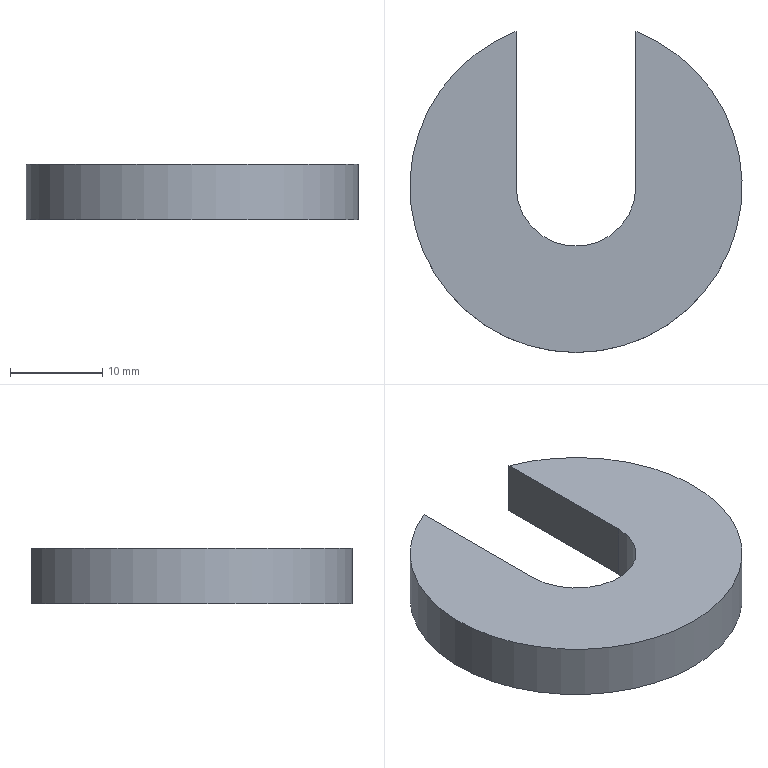Component | NX | C_WASHER | 1 solid | 6 faces | box 36 x 34.79 x 6 mm | volume 4336 mm3 | plane 4 | cylinder 2 | commonest cylinder face diameters 36 x1 13 x1
STEP:
#1=CARTESIAN_POINT('',(0.,0.,0.));
#2=DIRECTION('',(0.,0.,1.));
#3=DIRECTION('',(1.,0.,0.));
#4=AXIS2_PLACEMENT_3D('',#1,#2,#3);
#5=CARTESIAN_POINT('',(-6.5,16.785,22.));
#6=VERTEX_POINT('',#5);
#7=CARTESIAN_POINT('',(6.5,16.785,22.));
#8=VERTEX_POINT('',#7);
#9=CARTESIAN_POINT('',(0.,0.,22.));
#10=DIRECTION('',(0.,0.,1.));
#11=DIRECTION('',(0.,-1.,0.));
#12=AXIS2_PLACEMENT_3D('',#9,#10,#11);
#13=CIRCLE('',#12,18.);
#14=CARTESIAN_POINT('',(0.,0.,28.));
#15=DIRECTION('',(0.,0.,-1.));
#16=DIRECTION('',(0.,1.,0.));
#17=AXIS2_PLACEMENT_3D('',#14,#15,#16);
#18=CYLINDRICAL_SURFACE('',#17,18.);
#19=CARTESIAN_POINT('',(9.425,6.));
#20=DIRECTION('',(-1.,0.));
#21=VECTOR('',#20,1.);
#22=LINE('',#19,#21);
#23=(GEOMETRIC_REPRESENTATION_CONTEXT(2)PARAMETRIC_REPRESENTATION_CONTEXT()REPRESENTATION_CONTEXT('',''));
#24=DEFINITIONAL_REPRESENTATION('',(#22),#23);
#25=PCURVE('',#18,#24);
#26=CARTESIAN_POINT('',(0.,0.,22.));
#27=DIRECTION('',(0.,0.,1.));
#28=DIRECTION('',(0.,-1.,0.));
#29=AXIS2_PLACEMENT_3D('',#26,#27,#28);
#30=PLANE('',#29);
#31=CARTESIAN_POINT('',(0.,0.));
#32=DIRECTION('',(1.,0.));
#33=AXIS2_PLACEMENT_2D('',#31,#32);
#34=CIRCLE('',#33,18.);
#35=(GEOMETRIC_REPRESENTATION_CONTEXT(2)PARAMETRIC_REPRESENTATION_CONTEXT()REPRESENTATION_CONTEXT('',''));
#36=DEFINITIONAL_REPRESENTATION('',(#34),#35);
#37=PCURVE('',#30,#36);
#38=SURFACE_CURVE('',#13,(#25,#37),.PCURVE_S1.);
#39=EDGE_CURVE('',#6,#8,#38,.T.);
#40=ORIENTED_EDGE('',*,*,#39,.T.);
#41=CARTESIAN_POINT('',(6.5,16.785,28.));
#42=VERTEX_POINT('',#41);
#43=CARTESIAN_POINT('',(6.5,16.785,28.));
#44=DIRECTION('',(0.,0.,-1.));
#45=VECTOR('',#44,1.);
#46=LINE('',#43,#45);
#47=CARTESIAN_POINT('',(0.3695,0.));
#48=DIRECTION('',(0.,1.));
#49=VECTOR('',#48,1.);
#50=LINE('',#47,#49);
#51=(GEOMETRIC_REPRESENTATION_CONTEXT(2)PARAMETRIC_REPRESENTATION_CONTEXT()REPRESENTATION_CONTEXT('',''));
#52=DEFINITIONAL_REPRESENTATION('',(#50),#51);
#53=PCURVE('',#18,#52);
#54=CARTESIAN_POINT('',(6.5,16.785,28.));
#55=DIRECTION('',(1.,0.,0.));
#56=DIRECTION('',(0.,0.,1.));
#57=AXIS2_PLACEMENT_3D('',#54,#55,#56);
#58=PLANE('',#57);
#59=CARTESIAN_POINT('',(0.,0.));
#60=DIRECTION('',(-1.,0.));
#61=VECTOR('',#60,1.);
#62=LINE('',#59,#61);
#63=(GEOMETRIC_REPRESENTATION_CONTEXT(2)PARAMETRIC_REPRESENTATION_CONTEXT()REPRESENTATION_CONTEXT('',''));
#64=DEFINITIONAL_REPRESENTATION('',(#62),#63);
#65=PCURVE('',#58,#64);
#66=SURFACE_CURVE('',#46,(#53,#65),.PCURVE_S1.);
#67=EDGE_CURVE('',#42,#8,#66,.T.);
#68=ORIENTED_EDGE('',*,*,#67,.F.);
#69=CARTESIAN_POINT('',(-6.5,16.785,28.));
#70=VERTEX_POINT('',#69);
#71=CARTESIAN_POINT('',(0.,0.,28.));
#72=DIRECTION('',(0.,0.,1.));
#73=DIRECTION('',(0.,-1.,0.));
#74=AXIS2_PLACEMENT_3D('',#71,#72,#73);
#75=CIRCLE('',#74,18.);
#76=CARTESIAN_POINT('',(9.425,0.));
#77=DIRECTION('',(-1.,0.));
#78=VECTOR('',#77,1.);
#79=LINE('',#76,#78);
#80=(GEOMETRIC_REPRESENTATION_CONTEXT(2)PARAMETRIC_REPRESENTATION_CONTEXT()REPRESENTATION_CONTEXT('',''));
#81=DEFINITIONAL_REPRESENTATION('',(#79),#80);
#82=PCURVE('',#18,#81);
#83=CARTESIAN_POINT('',(0.,0.,28.));
#84=DIRECTION('',(0.,0.,1.));
#85=DIRECTION('',(0.,-1.,0.));
#86=AXIS2_PLACEMENT_3D('',#83,#84,#85);
#87=PLANE('',#86);
#88=CARTESIAN_POINT('',(0.,0.));
#89=DIRECTION('',(1.,0.));
#90=AXIS2_PLACEMENT_2D('',#88,#89);
#91=CIRCLE('',#90,18.);
#92=(GEOMETRIC_REPRESENTATION_CONTEXT(2)PARAMETRIC_REPRESENTATION_CONTEXT()REPRESENTATION_CONTEXT('',''));
#93=DEFINITIONAL_REPRESENTATION('',(#91),#92);
#94=PCURVE('',#87,#93);
#95=SURFACE_CURVE('',#75,(#82,#94),.PCURVE_S1.);
#96=EDGE_CURVE('',#70,#42,#95,.T.);
#97=ORIENTED_EDGE('',*,*,#96,.F.);
#98=CARTESIAN_POINT('',(-6.5,16.785,28.));
#99=DIRECTION('',(0.,0.,-1.));
#100=VECTOR('',#99,1.);
#101=LINE('',#98,#100);
#102=CARTESIAN_POINT('',(5.914,0.));
#103=DIRECTION('',(0.,1.));
#104=VECTOR('',#103,1.);
#105=LINE('',#102,#104);
#106=(GEOMETRIC_REPRESENTATION_CONTEXT(2)PARAMETRIC_REPRESENTATION_CONTEXT()REPRESENTATION_CONTEXT('',''));
#107=DEFINITIONAL_REPRESENTATION('',(#105),#106);
#108=PCURVE('',#18,#107);
#109=CARTESIAN_POINT('',(-6.5,0.,28.));
#110=DIRECTION('',(-1.,0.,0.));
#111=DIRECTION('',(0.,0.,-1.));
#112=AXIS2_PLACEMENT_3D('',#109,#110,#111);
#113=PLANE('',#112);
#114=CARTESIAN_POINT('',(0.,-16.785));
#115=DIRECTION('',(1.,0.));
#116=VECTOR('',#115,1.);
#117=LINE('',#114,#116);
#118=(GEOMETRIC_REPRESENTATION_CONTEXT(2)PARAMETRIC_REPRESENTATION_CONTEXT()REPRESENTATION_CONTEXT('',''));
#119=DEFINITIONAL_REPRESENTATION('',(#117),#118);
#120=PCURVE('',#113,#119);
#121=SURFACE_CURVE('',#101,(#108,#120),.PCURVE_S1.);
#122=EDGE_CURVE('',#70,#6,#121,.T.);
#123=ORIENTED_EDGE('',*,*,#122,.T.);
#124=EDGE_LOOP('',(#40,#68,#97,#123));
#125=FACE_BOUND('',#124,.T.);
#126=ADVANCED_FACE('',(#125),#18,.T.);
#127=CARTESIAN_POINT('',(6.5,0.,22.));
#128=VERTEX_POINT('',#127);
#129=CARTESIAN_POINT('',(6.5,16.785,22.));
#130=DIRECTION('',(0.,-1.,0.));
#131=VECTOR('',#130,1.);
#132=LINE('',#129,#131);
#133=CARTESIAN_POINT('',(-6.,0.));
#134=DIRECTION('',(0.,1.));
#135=VECTOR('',#134,1.);
#136=LINE('',#133,#135);
#137=(GEOMETRIC_REPRESENTATION_CONTEXT(2)PARAMETRIC_REPRESENTATION_CONTEXT()REPRESENTATION_CONTEXT('',''));
#138=DEFINITIONAL_REPRESENTATION('',(#136),#137);
#139=PCURVE('',#58,#138);
#140=CARTESIAN_POINT('',(-16.785,6.5));
#141=DIRECTION('',(1.,0.));
#142=VECTOR('',#141,1.);
#143=LINE('',#140,#142);
#144=(GEOMETRIC_REPRESENTATION_CONTEXT(2)PARAMETRIC_REPRESENTATION_CONTEXT()REPRESENTATION_CONTEXT('',''));
#145=DEFINITIONAL_REPRESENTATION('',(#143),#144);
#146=PCURVE('',#30,#145);
#147=SURFACE_CURVE('',#132,(#139,#146),.PCURVE_S1.);
#148=EDGE_CURVE('',#8,#128,#147,.T.);
#149=ORIENTED_EDGE('',*,*,#148,.T.);
#150=CARTESIAN_POINT('',(6.5,0.,28.));
#151=VERTEX_POINT('',#150);
#152=CARTESIAN_POINT('',(6.5,0.,28.));
#153=DIRECTION('',(0.,0.,-1.));
#154=VECTOR('',#153,1.);
#155=LINE('',#152,#154);
#156=CARTESIAN_POINT('',(0.,16.785));
#157=DIRECTION('',(-1.,0.));
#158=VECTOR('',#157,1.);
#159=LINE('',#156,#158);
#160=(GEOMETRIC_REPRESENTATION_CONTEXT(2)PARAMETRIC_REPRESENTATION_CONTEXT()REPRESENTATION_CONTEXT('',''));
#161=DEFINITIONAL_REPRESENTATION('',(#159),#160);
#162=PCURVE('',#58,#161);
#163=CARTESIAN_POINT('',(0.,0.,28.));
#164=DIRECTION('',(0.,0.,-1.));
#165=DIRECTION('',(0.,1.,0.));
#166=AXIS2_PLACEMENT_3D('',#163,#164,#165);
#167=CYLINDRICAL_SURFACE('',#166,6.5);
#168=CARTESIAN_POINT('',(1.571,0.));
#169=DIRECTION('',(0.,1.));
#170=VECTOR('',#169,1.);
#171=LINE('',#168,#170);
#172=(GEOMETRIC_REPRESENTATION_CONTEXT(2)PARAMETRIC_REPRESENTATION_CONTEXT()REPRESENTATION_CONTEXT('',''));
#173=DEFINITIONAL_REPRESENTATION('',(#171),#172);
#174=PCURVE('',#167,#173);
#175=SURFACE_CURVE('',#155,(#162,#174),.PCURVE_S1.);
#176=EDGE_CURVE('',#151,#128,#175,.T.);
#177=ORIENTED_EDGE('',*,*,#176,.F.);
#178=CARTESIAN_POINT('',(6.5,16.785,28.));
#179=DIRECTION('',(0.,-1.,0.));
#180=VECTOR('',#179,1.);
#181=LINE('',#178,#180);
#182=CARTESIAN_POINT('',(0.,0.));
#183=DIRECTION('',(0.,1.));
#184=VECTOR('',#183,1.);
#185=LINE('',#182,#184);
#186=(GEOMETRIC_REPRESENTATION_CONTEXT(2)PARAMETRIC_REPRESENTATION_CONTEXT()REPRESENTATION_CONTEXT('',''));
#187=DEFINITIONAL_REPRESENTATION('',(#185),#186);
#188=PCURVE('',#58,#187);
#189=CARTESIAN_POINT('',(-16.785,6.5));
#190=DIRECTION('',(1.,0.));
#191=VECTOR('',#190,1.);
#192=LINE('',#189,#191);
#193=(GEOMETRIC_REPRESENTATION_CONTEXT(2)PARAMETRIC_REPRESENTATION_CONTEXT()REPRESENTATION_CONTEXT('',''));
#194=DEFINITIONAL_REPRESENTATION('',(#192),#193);
#195=PCURVE('',#87,#194);
#196=SURFACE_CURVE('',#181,(#188,#195),.PCURVE_S1.);
#197=EDGE_CURVE('',#42,#151,#196,.T.);
#198=ORIENTED_EDGE('',*,*,#197,.F.);
#199=ORIENTED_EDGE('',*,*,#67,.T.);
#200=EDGE_LOOP('',(#149,#177,#198,#199));
#201=FACE_BOUND('',#200,.T.);
#202=ADVANCED_FACE('',(#201),#58,.F.);
#203=ORIENTED_EDGE('',*,*,#176,.F.);
#204=CARTESIAN_POINT('',(-6.5,-0.,28.));
#205=VERTEX_POINT('',#204);
#206=CARTESIAN_POINT('',(0.,0.,28.));
#207=DIRECTION('',(0.,0.,-1.));
#208=DIRECTION('',(0.,-1.,0.));
#209=AXIS2_PLACEMENT_3D('',#206,#207,#208);
#210=CIRCLE('',#209,6.5);
#211=CARTESIAN_POINT('',(-3.142,0.));
#212=DIRECTION('',(1.,0.));
#213=VECTOR('',#212,1.);
#214=LINE('',#211,#213);
#215=(GEOMETRIC_REPRESENTATION_CONTEXT(2)PARAMETRIC_REPRESENTATION_CONTEXT()REPRESENTATION_CONTEXT('',''));
#216=DEFINITIONAL_REPRESENTATION('',(#214),#215);
#217=PCURVE('',#167,#216);
#218=CARTESIAN_POINT('',(6.5,0.));
#219=CARTESIAN_POINT('',(6.5,-11.258));
#220=CARTESIAN_POINT('',(-3.25,-5.629));
#221=CARTESIAN_POINT('',(-13.,-0.));
#222=CARTESIAN_POINT('',(-3.25,5.629));
#223=CARTESIAN_POINT('',(6.5,11.258));
#224=CARTESIAN_POINT('',(6.5,0.));
#225=(BOUNDED_CURVE()B_SPLINE_CURVE(2,(#218,#219,#220,#221,#222,#223,#224),.UNSPECIFIED.,.T.,.F.)B_SPLINE_CURVE_WITH_KNOTS((1,2,2,2,2,1),(-2.094,0.,2.094,4.189,6.283,8.378),.UNSPECIFIED.)CURVE()GEOMETRIC_REPRESENTATION_ITEM()RATIONAL_B_SPLINE_CURVE((1.,0.5,1.,0.5,1.,0.5,1.))REPRESENTATION_ITEM(''));
#226=(GEOMETRIC_REPRESENTATION_CONTEXT(2)PARAMETRIC_REPRESENTATION_CONTEXT()REPRESENTATION_CONTEXT('',''));
#227=DEFINITIONAL_REPRESENTATION('',(#225),#226);
#228=PCURVE('',#87,#227);
#229=SURFACE_CURVE('',#210,(#217,#228),.PCURVE_S1.);
#230=EDGE_CURVE('',#151,#205,#229,.T.);
#231=ORIENTED_EDGE('',*,*,#230,.T.);
#232=CARTESIAN_POINT('',(-6.5,-0.,22.));
#233=VERTEX_POINT('',#232);
#234=CARTESIAN_POINT('',(-6.5,-0.,28.));
#235=DIRECTION('',(0.,0.,-1.));
#236=VECTOR('',#235,1.);
#237=LINE('',#234,#236);
#238=CARTESIAN_POINT('',(4.712,0.));
#239=DIRECTION('',(0.,1.));
#240=VECTOR('',#239,1.);
#241=LINE('',#238,#240);
#242=(GEOMETRIC_REPRESENTATION_CONTEXT(2)PARAMETRIC_REPRESENTATION_CONTEXT()REPRESENTATION_CONTEXT('',''));
#243=DEFINITIONAL_REPRESENTATION('',(#241),#242);
#244=PCURVE('',#167,#243);
#245=CARTESIAN_POINT('',(0.,0.));
#246=DIRECTION('',(1.,0.));
#247=VECTOR('',#246,1.);
#248=LINE('',#245,#247);
#249=(GEOMETRIC_REPRESENTATION_CONTEXT(2)PARAMETRIC_REPRESENTATION_CONTEXT()REPRESENTATION_CONTEXT('',''));
#250=DEFINITIONAL_REPRESENTATION('',(#248),#249);
#251=PCURVE('',#113,#250);
#252=SURFACE_CURVE('',#237,(#244,#251),.PCURVE_S1.);
#253=EDGE_CURVE('',#205,#233,#252,.T.);
#254=ORIENTED_EDGE('',*,*,#253,.T.);
#255=CARTESIAN_POINT('',(0.,0.,22.));
#256=DIRECTION('',(0.,0.,-1.));
#257=DIRECTION('',(0.,-1.,0.));
#258=AXIS2_PLACEMENT_3D('',#255,#256,#257);
#259=CIRCLE('',#258,6.5);
#260=CARTESIAN_POINT('',(-3.142,6.));
#261=DIRECTION('',(1.,0.));
#262=VECTOR('',#261,1.);
#263=LINE('',#260,#262);
#264=(GEOMETRIC_REPRESENTATION_CONTEXT(2)PARAMETRIC_REPRESENTATION_CONTEXT()REPRESENTATION_CONTEXT('',''));
#265=DEFINITIONAL_REPRESENTATION('',(#263),#264);
#266=PCURVE('',#167,#265);
#267=CARTESIAN_POINT('',(6.5,0.));
#268=CARTESIAN_POINT('',(6.5,-11.258));
#269=CARTESIAN_POINT('',(-3.25,-5.629));
#270=CARTESIAN_POINT('',(-13.,-0.));
#271=CARTESIAN_POINT('',(-3.25,5.629));
#272=CARTESIAN_POINT('',(6.5,11.258));
#273=CARTESIAN_POINT('',(6.5,0.));
#274=(BOUNDED_CURVE()B_SPLINE_CURVE(2,(#267,#268,#269,#270,#271,#272,#273),.UNSPECIFIED.,.T.,.F.)B_SPLINE_CURVE_WITH_KNOTS((1,2,2,2,2,1),(-2.094,0.,2.094,4.189,6.283,8.378),.UNSPECIFIED.)CURVE()GEOMETRIC_REPRESENTATION_ITEM()RATIONAL_B_SPLINE_CURVE((1.,0.5,1.,0.5,1.,0.5,1.))REPRESENTATION_ITEM(''));
#275=(GEOMETRIC_REPRESENTATION_CONTEXT(2)PARAMETRIC_REPRESENTATION_CONTEXT()REPRESENTATION_CONTEXT('',''));
#276=DEFINITIONAL_REPRESENTATION('',(#274),#275);
#277=PCURVE('',#30,#276);
#278=SURFACE_CURVE('',#259,(#266,#277),.PCURVE_S1.);
#279=EDGE_CURVE('',#128,#233,#278,.T.);
#280=ORIENTED_EDGE('',*,*,#279,.F.);
#281=EDGE_LOOP('',(#203,#231,#254,#280));
#282=FACE_BOUND('',#281,.F.);
#283=ADVANCED_FACE('',(#282),#167,.F.);
#284=CARTESIAN_POINT('',(-6.5,0.,22.));
#285=DIRECTION('',(0.,1.,0.));
#286=VECTOR('',#285,1.);
#287=LINE('',#284,#286);
#288=CARTESIAN_POINT('',(6.,0.));
#289=DIRECTION('',(0.,-1.));
#290=VECTOR('',#289,1.);
#291=LINE('',#288,#290);
#292=(GEOMETRIC_REPRESENTATION_CONTEXT(2)PARAMETRIC_REPRESENTATION_CONTEXT()REPRESENTATION_CONTEXT('',''));
#293=DEFINITIONAL_REPRESENTATION('',(#291),#292);
#294=PCURVE('',#113,#293);
#295=CARTESIAN_POINT('',(0.,-6.5));
#296=DIRECTION('',(-1.,0.));
#297=VECTOR('',#296,1.);
#298=LINE('',#295,#297);
#299=(GEOMETRIC_REPRESENTATION_CONTEXT(2)PARAMETRIC_REPRESENTATION_CONTEXT()REPRESENTATION_CONTEXT('',''));
#300=DEFINITIONAL_REPRESENTATION('',(#298),#299);
#301=PCURVE('',#30,#300);
#302=SURFACE_CURVE('',#287,(#294,#301),.PCURVE_S1.);
#303=EDGE_CURVE('',#233,#6,#302,.T.);
#304=ORIENTED_EDGE('',*,*,#303,.T.);
#305=ORIENTED_EDGE('',*,*,#122,.F.);
#306=CARTESIAN_POINT('',(-6.5,0.,28.));
#307=DIRECTION('',(0.,1.,0.));
#308=VECTOR('',#307,1.);
#309=LINE('',#306,#308);
#310=CARTESIAN_POINT('',(0.,0.));
#311=DIRECTION('',(0.,-1.));
#312=VECTOR('',#311,1.);
#313=LINE('',#310,#312);
#314=(GEOMETRIC_REPRESENTATION_CONTEXT(2)PARAMETRIC_REPRESENTATION_CONTEXT()REPRESENTATION_CONTEXT('',''));
#315=DEFINITIONAL_REPRESENTATION('',(#313),#314);
#316=PCURVE('',#113,#315);
#317=CARTESIAN_POINT('',(0.,-6.5));
#318=DIRECTION('',(-1.,0.));
#319=VECTOR('',#318,1.);
#320=LINE('',#317,#319);
#321=(GEOMETRIC_REPRESENTATION_CONTEXT(2)PARAMETRIC_REPRESENTATION_CONTEXT()REPRESENTATION_CONTEXT('',''));
#322=DEFINITIONAL_REPRESENTATION('',(#320),#321);
#323=PCURVE('',#87,#322);
#324=SURFACE_CURVE('',#309,(#316,#323),.PCURVE_S1.);
#325=EDGE_CURVE('',#205,#70,#324,.T.);
#326=ORIENTED_EDGE('',*,*,#325,.F.);
#327=ORIENTED_EDGE('',*,*,#253,.T.);
#328=EDGE_LOOP('',(#304,#305,#326,#327));
#329=FACE_BOUND('',#328,.T.);
#330=ADVANCED_FACE('',(#329),#113,.F.);
#331=ORIENTED_EDGE('',*,*,#96,.T.);
#332=ORIENTED_EDGE('',*,*,#197,.T.);
#333=ORIENTED_EDGE('',*,*,#230,.T.);
#334=ORIENTED_EDGE('',*,*,#325,.T.);
#335=EDGE_LOOP('',(#331,#332,#333,#334));
#336=FACE_BOUND('',#335,.T.);
#337=ADVANCED_FACE('',(#336),#87,.T.);
#338=ORIENTED_EDGE('',*,*,#39,.F.);
#339=ORIENTED_EDGE('',*,*,#303,.F.);
#340=ORIENTED_EDGE('',*,*,#279,.F.);
#341=ORIENTED_EDGE('',*,*,#148,.F.);
#342=EDGE_LOOP('',(#338,#339,#340,#341));
#343=FACE_BOUND('',#342,.T.);
#344=ADVANCED_FACE('',(#343),#30,.F.);
#345=CLOSED_SHELL('',(#126,#202,#283,#330,#337,#344));
#346=MANIFOLD_SOLID_BREP('',#345);
#347=(LENGTH_UNIT()NAMED_UNIT(*)SI_UNIT(.MILLI.,.METRE.));
#348=UNCERTAINTY_MEASURE_WITH_UNIT(LENGTH_MEASURE(0.0000001),#347,'','');
#349=(NAMED_UNIT(*)PLANE_ANGLE_UNIT()SI_UNIT($,.RADIAN.));
#350=(NAMED_UNIT(*)SI_UNIT($,.STERADIAN.)SOLID_ANGLE_UNIT());
#351=(GEOMETRIC_REPRESENTATION_CONTEXT(3)GLOBAL_UNCERTAINTY_ASSIGNED_CONTEXT((#348))GLOBAL_UNIT_ASSIGNED_CONTEXT((#347,#349,#350))REPRESENTATION_CONTEXT('',''));
#352=ADVANCED_BREP_SHAPE_REPRESENTATION('',(#4,#346),#351);